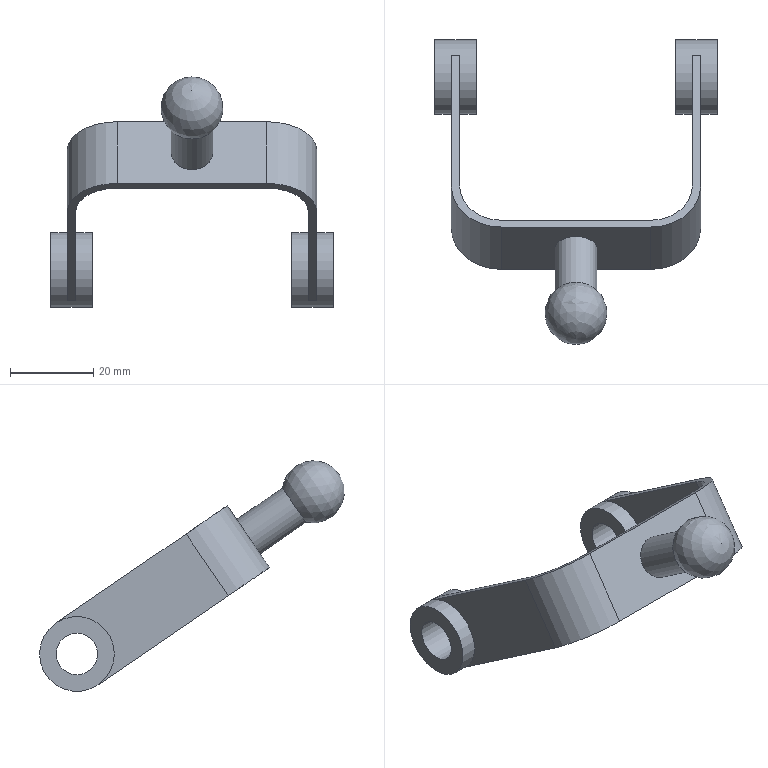Component | NX | 3 | 2 solids | 24 faces | volume 10870 mm3 | plane 13 | cylinder 10 | sphere 1 | commonest cylinder face diameters 10 x4 24 x2 20 x2 18 x2